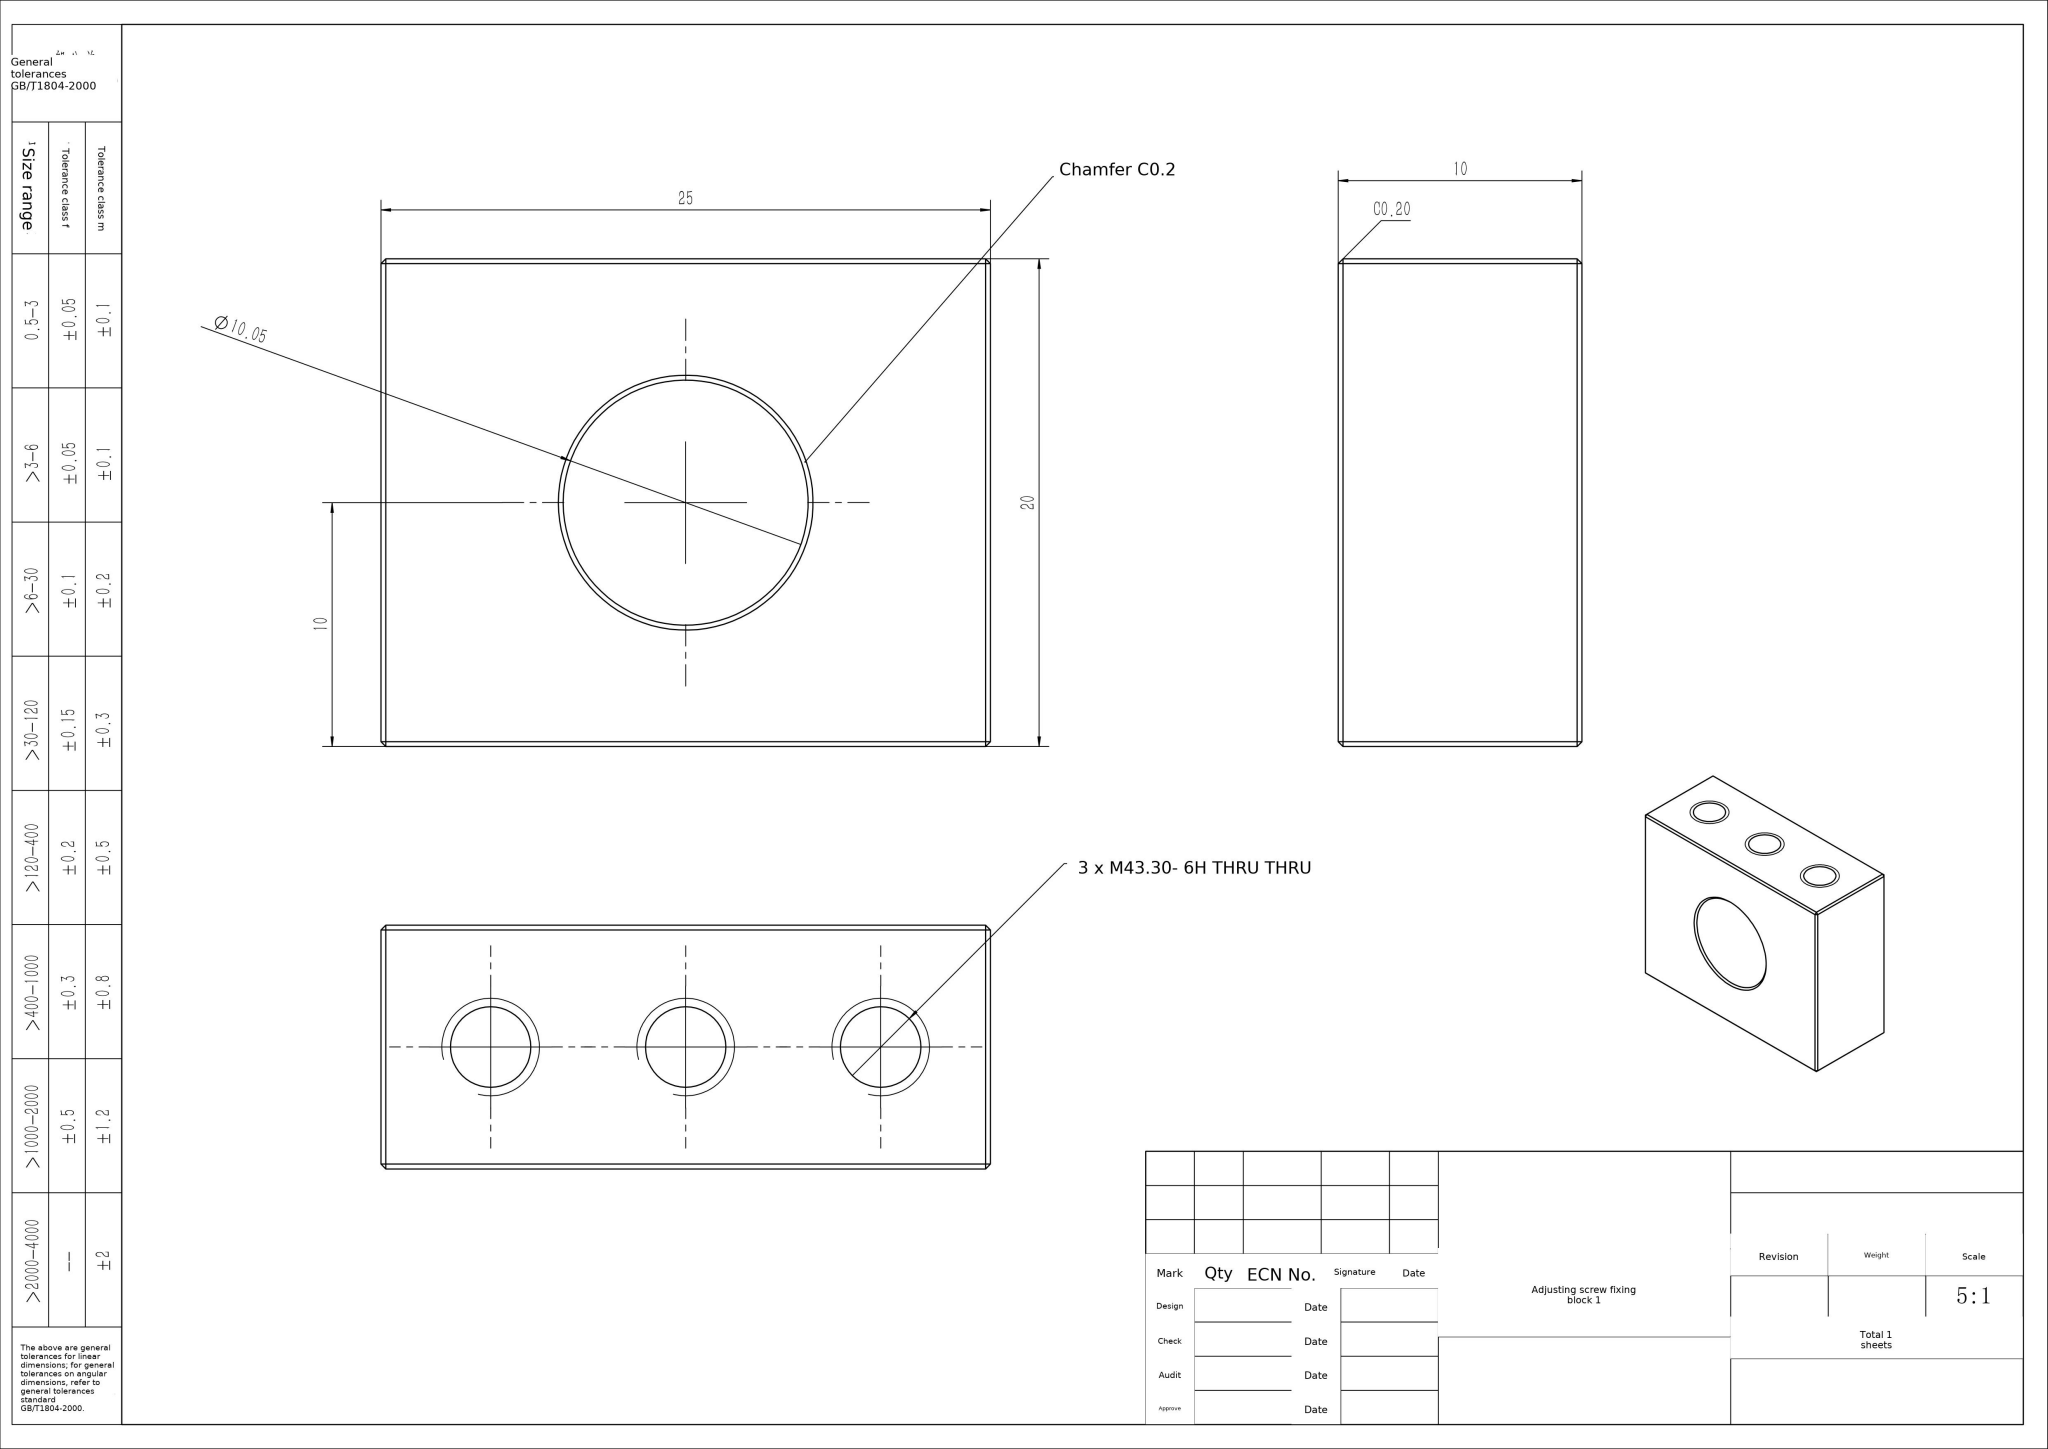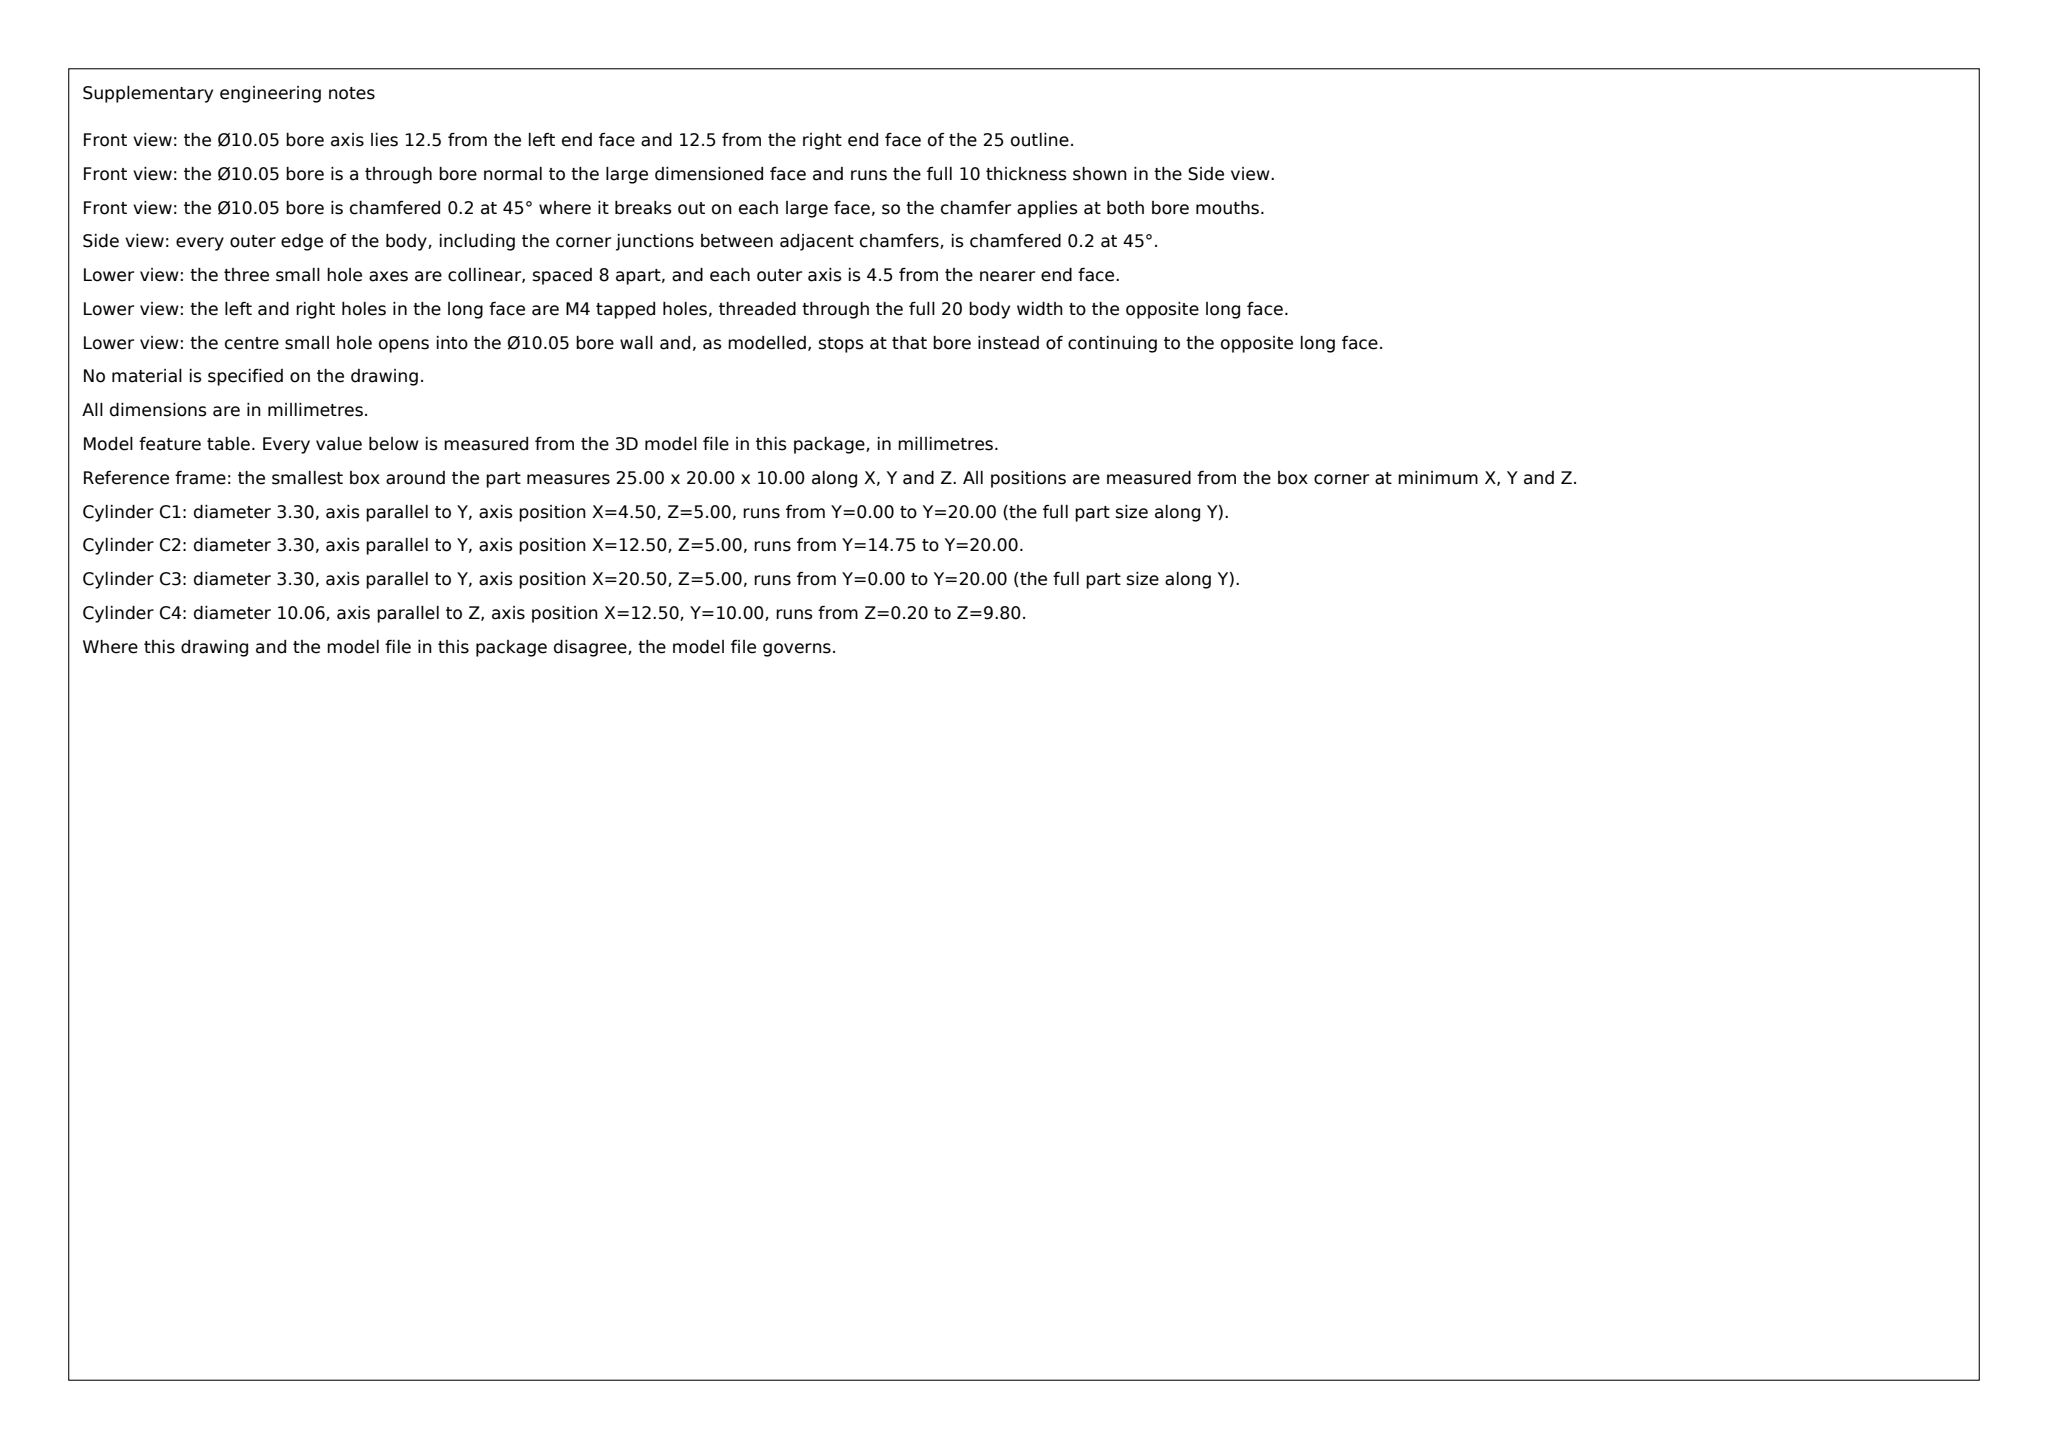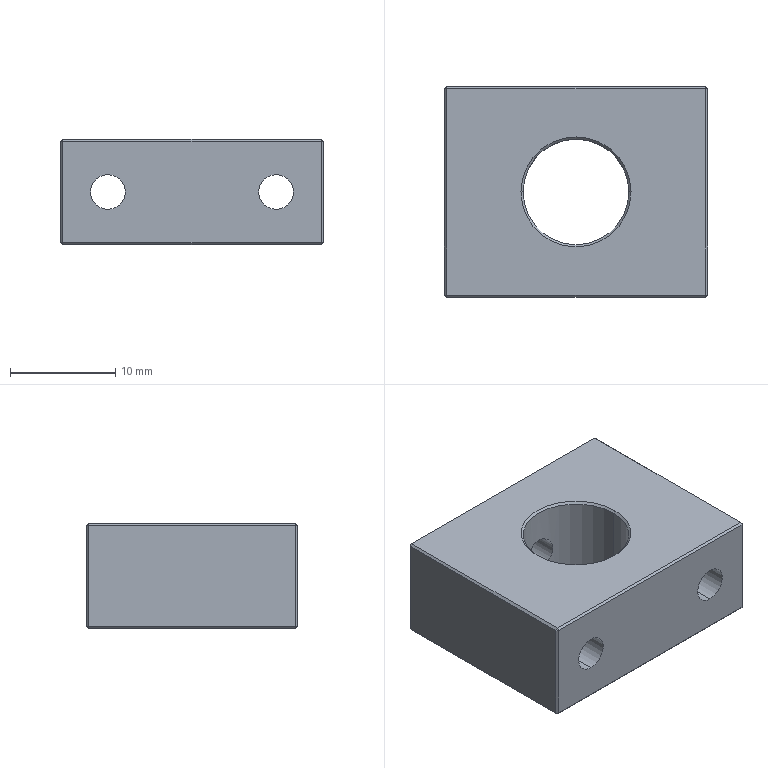Part | SolidWorks | mm | 1 solid | 38 faces | box 25 x 20 x 10 mm | volume 3816 mm3 | plane 26 | cylinder 8 | cone 4 | commonest cylinder face diameters 3.3 x6 10.05 x2
Drawing notes:
Ø10.05 THRU: 12.5 FROM EA 25 END (ON CL), 10 UP FROM BTM | from the solid: cyl dia 10.05 axis z at (x=12.5, y=10.0), bbox 25x20x10
3 x M4 THRU: 4.5 FROM EA END, 2 x 8 EQL SP, CL OF 25 | from the solid: cyl dia 3.3 axis y at x=4.5, 12.5, 20.5; bbox x=25
3 x M4 AXES 5 FROM FACE = MID OF 10 THK | from the solid: cyl dia 3.3 axis y at z=5.0; bbox z=10
C0.2 = 90° CSK TO Ø10.45 BOTH ENDS OF Ø10.05 BORE | from the solid: cones 90° incl, ref dia 10.45 & 10.05, qty 2; bore length 9.6 in 10 thk
build123d program:
from build123d import *

# Parameters (mm, degrees)
SKETCH1_W              = 25
SKETCH1_H              = 10
BOSS_EXTRUDE1_DEPTH    = 10
SKETCH3_R              = 5.025
CUT_EXTRUDE1_DEPTH     = 19.875
M4_TAPPED_HOLE1_REACH  = 26.109
M4_TAPPED_HOLE1_BORE_R = 1.65
CHAMFER1_SIZE          = 0.2


with BuildPart() as part:
    # Sketch1 → Boss-Extrude1 (new, symmetric)
    with BuildSketch(Plane(origin=(0, 0, 0), x_dir=(1, 0, 0), z_dir=(0, 1, 0))):
        Rectangle(SKETCH1_W, SKETCH1_H)
    extrude(amount=BOSS_EXTRUDE1_DEPTH, both=True)

    # Sketch3 → Cut-Extrude1 (cut, through all)
    with BuildSketch(Plane.XY.offset(5)):
        Circle(SKETCH3_R)
    extrude(amount=-CUT_EXTRUDE1_DEPTH, mode=Mode.SUBTRACT)

    # M4 Tapped Hole1 bore → M4 Tapped Hole1 (cut, up to next)
    with BuildSketch(Plane(origin=(0, 10, 0), x_dir=(1, 0, 0), z_dir=(0, 1, 0)), mode=Mode.PRIVATE) as m4_tapped_hole1_sk1:
        with Locations((-8, 0)):
            Circle(M4_TAPPED_HOLE1_BORE_R)
    m4_tapped_hole1_tool1 = extrude(m4_tapped_hole1_sk1.sketch, amount=-M4_TAPPED_HOLE1_REACH, mode=Mode.PRIVATE) & part.part
    # M4 Tapped Hole1 bore → M4 Tapped Hole1 (cut, up to next)
    with BuildSketch(Plane(origin=(0, 10, 0), x_dir=(1, 0, 0), z_dir=(0, 1, 0)), mode=Mode.PRIVATE) as m4_tapped_hole1_sk2:
        with Locations((8, 0)):
            Circle(M4_TAPPED_HOLE1_BORE_R)
    m4_tapped_hole1_tool2 = extrude(m4_tapped_hole1_sk2.sketch, amount=-M4_TAPPED_HOLE1_REACH, mode=Mode.PRIVATE) & part.part
    # M4 Tapped Hole1 bore → M4 Tapped Hole1 (cut, up to next)
    with BuildSketch(Plane(origin=(0, 10, 0), x_dir=(1, 0, 0), z_dir=(0, 1, 0)), mode=Mode.PRIVATE) as m4_tapped_hole1_sk3:
        Circle(M4_TAPPED_HOLE1_BORE_R)
    m4_tapped_hole1_tool3 = extrude(m4_tapped_hole1_sk3.sketch, amount=-M4_TAPPED_HOLE1_REACH, mode=Mode.PRIVATE) & part.part
    add(m4_tapped_hole1_tool1.solids().sort_by_distance((-8, 10, 0))[0], mode=Mode.SUBTRACT)
    add(m4_tapped_hole1_tool2.solids().sort_by_distance((8, 10, 0))[0], mode=Mode.SUBTRACT)
    add(m4_tapped_hole1_tool3.solids().sort_by_distance((0, 10, 0))[0], mode=Mode.SUBTRACT)

    # Chamfer1
    chamfer1_edges = [part.edges().sort_by_distance(p)[0] for p in [
        (-12.5, 10, 0),
        (-5.025, 0, -5),
        (-5.025, 0, 5),
        (0, 10, 5),
        (12.5, 10, 0),
        (0, -10, 5),
        (-12.5, -10, 0),
        (0, -10, -5),
        (12.5, -10, 0),
        (12.5, 0, 5),
        (-12.5, 0, 5),
        (-12.5, 0, -5),
        (12.5, 0, -5),
        (0, 10, -5),
    ]]
    chamfer(chamfer1_edges, length=CHAMFER1_SIZE)


solid = part.part